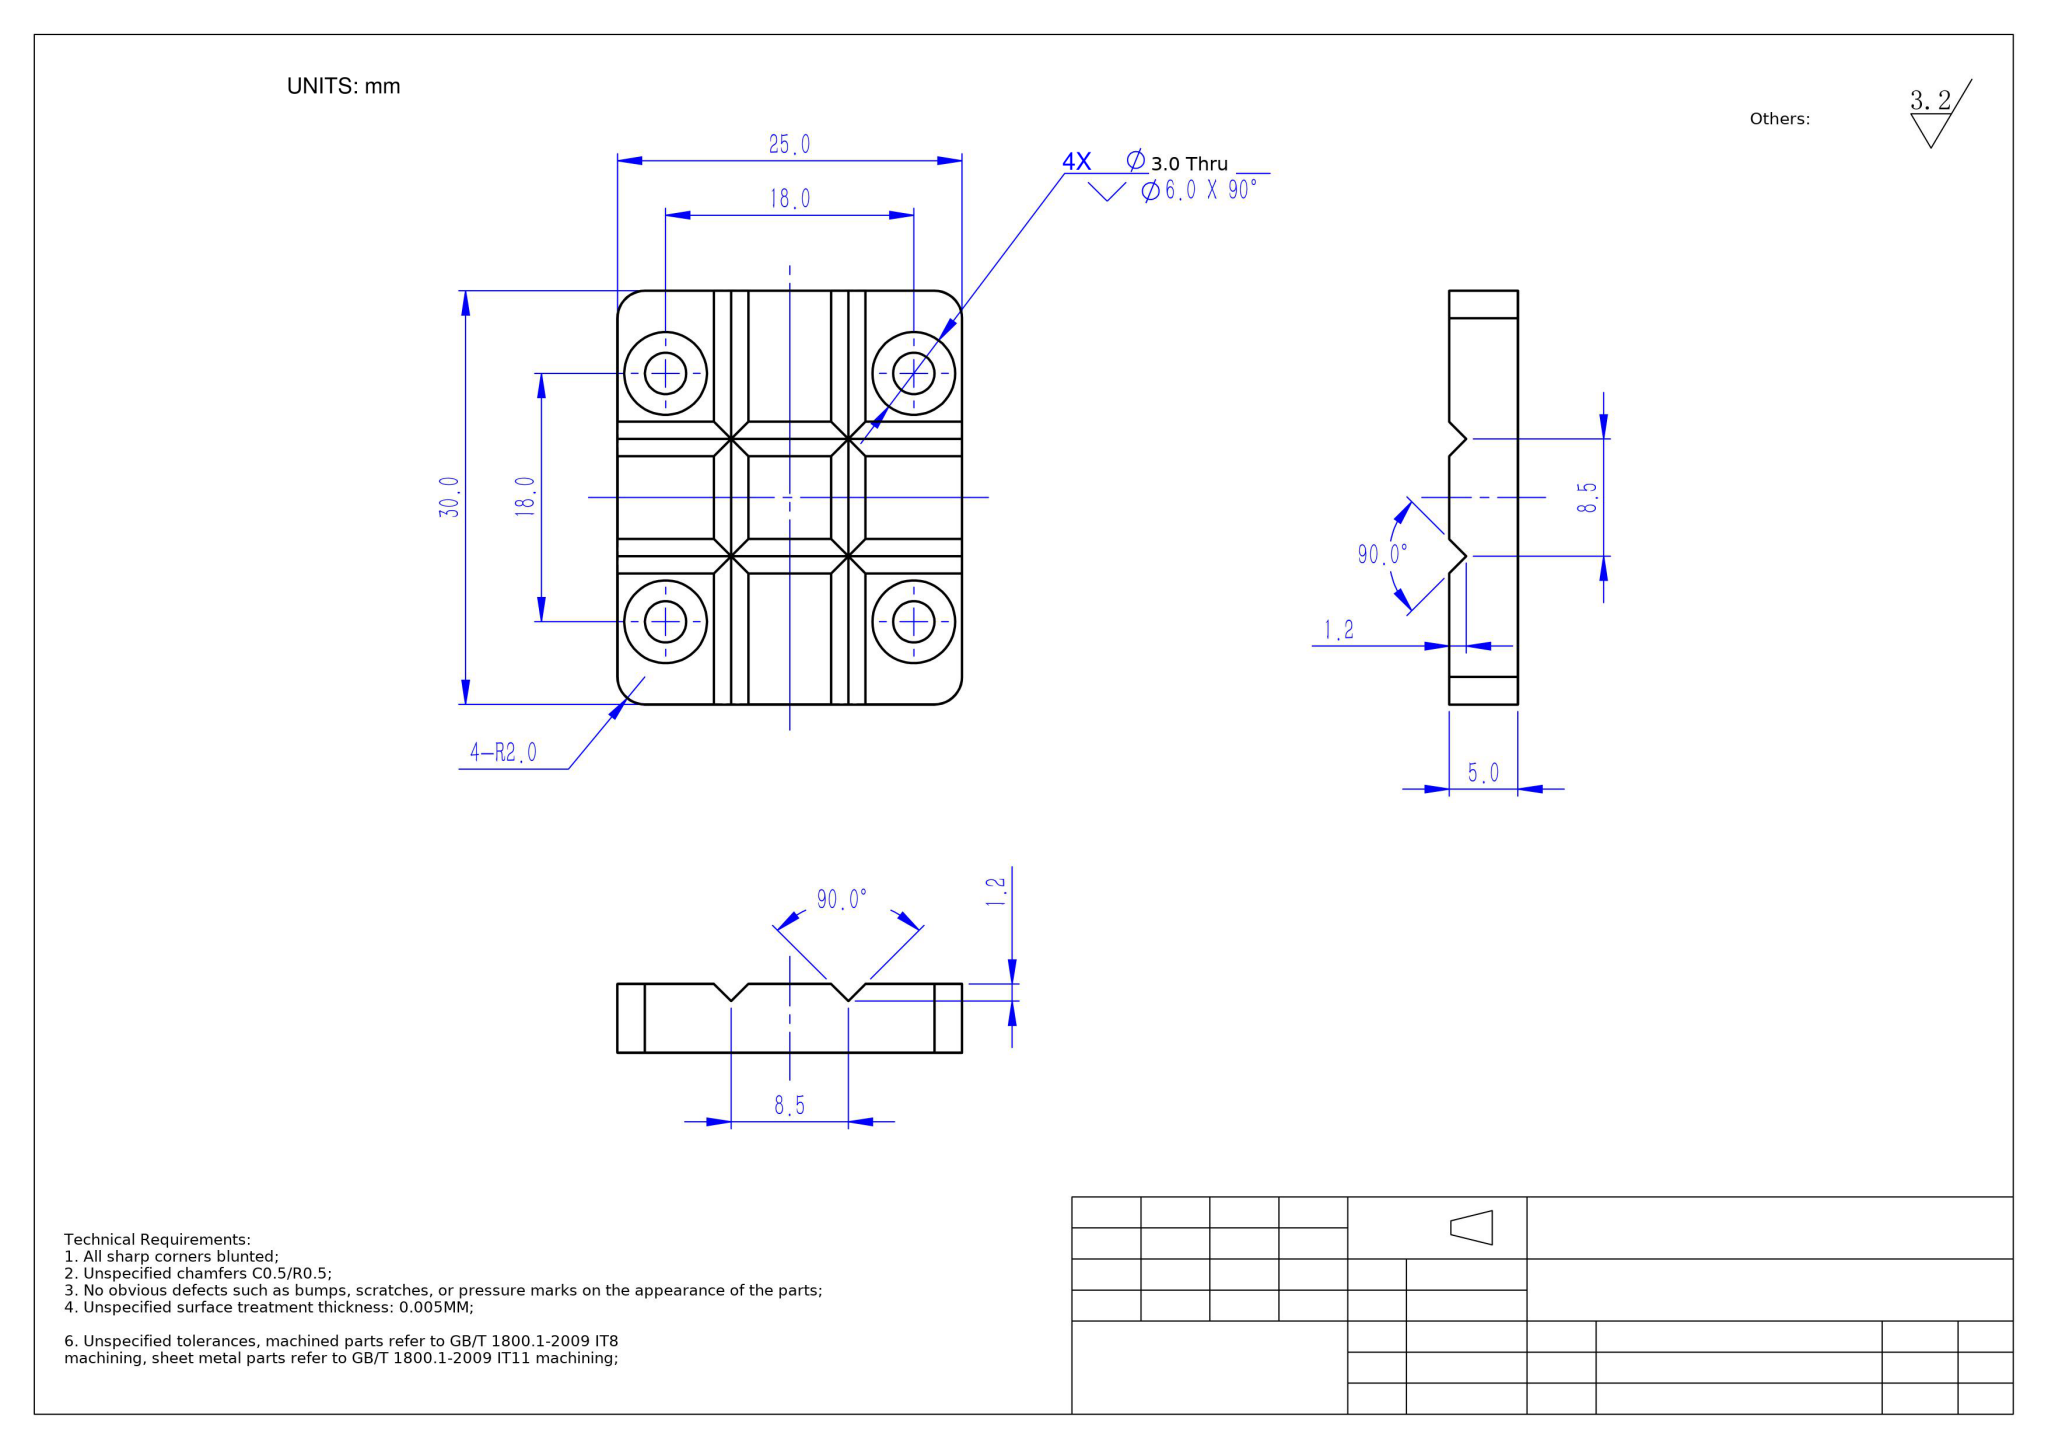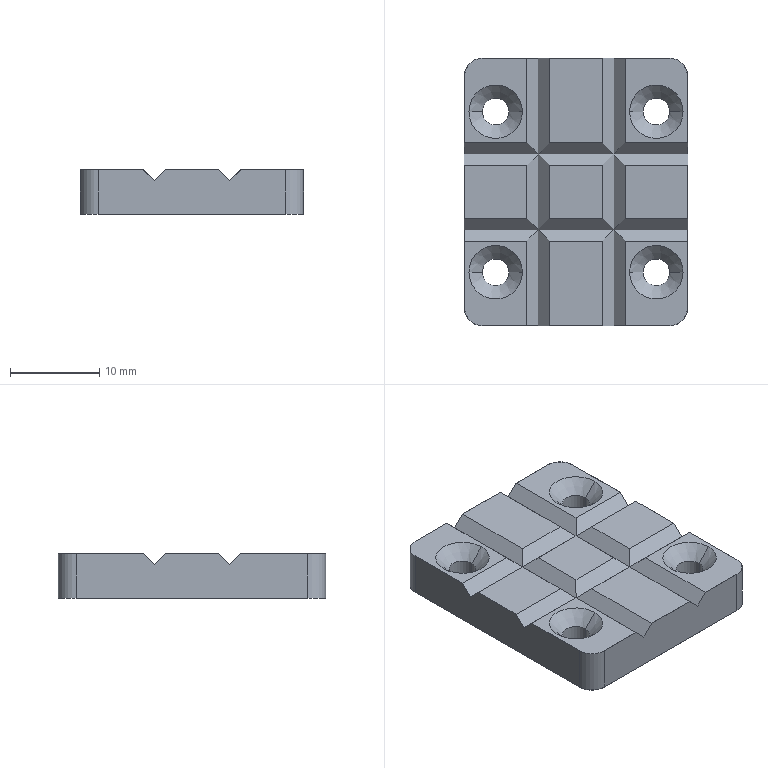Part | NX | mm | 1 solid | 82 faces | box 25 x 30 x 5 mm | volume 3373 mm3 | plane 54 | cone 16 | cylinder 12 | commonest cylinder face diameters 3 x8 4 x4